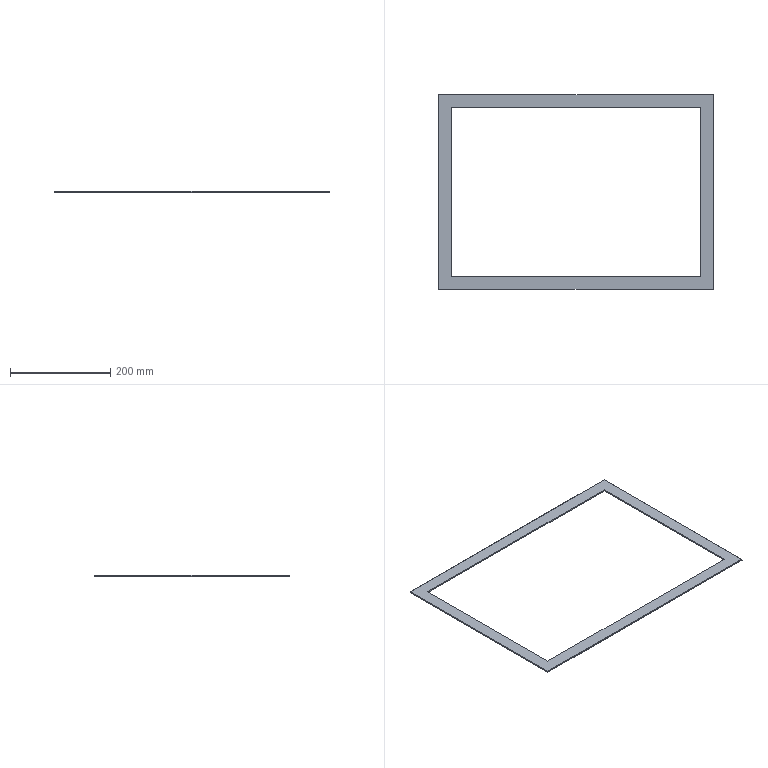Component | SolidWorks | LeftDoorPanelAssembly-1_WaterproofRubberStrip-1 | 1 solid | 18 faces | box 547.1 x 388.6 x 2.5 mm | volume 110544 mm3 | plane 18
build123d program:
from build123d import *

# Parameters (mm, degrees)
SKETCH1_W           = 547.1
SKETCH1_H           = 388.6
SKETCH1_W_2         = 497.1
SKETCH1_H_2         = 338.6
BOSS_EXTRUDE1_DEPTH = 2.5
CHAMFER1_SIZE       = 0.3


with BuildPart() as part:
    # Sketch1 → Boss-Extrude1 (new body)
    with BuildSketch(Plane.XY):
        Rectangle(SKETCH1_W, SKETCH1_H)
        Rectangle(SKETCH1_W_2, SKETCH1_H_2, mode=Mode.SUBTRACT)
    extrude(amount=BOSS_EXTRUDE1_DEPTH)

    # Chamfer1
    chamfer1_edges = [part.edges().sort_by_distance(p)[0] for p in [
        (273.55, 0, 2.5),
        (0, 194.3, 2.5),
        (-273.55, 0, 2.5),
        (0, 194.3, 0),
        (273.55, 0, 0),
        (0, -194.3, 0),
        (-273.55, 0, 0),
        (0, -194.3, 2.5),
    ]]
    chamfer(chamfer1_edges, length=CHAMFER1_SIZE)


solid = part.part

# Placed as in the assembly
solid = solid.moved(Location((235.358, 13.542, -71.9), (0, 0, 0)))
STEP:
#1=COLOUR_RGB('',0.7922,0.8196,0.9333);
#2=FILL_AREA_STYLE_COLOUR('',#1);
#3=FILL_AREA_STYLE('',(#2));
#4=SURFACE_STYLE_FILL_AREA(#3);
#5=SURFACE_SIDE_STYLE('',(#4));
#6=SURFACE_STYLE_USAGE(.BOTH.,#5);
#7=PRESENTATION_STYLE_ASSIGNMENT((#6));
#8=CARTESIAN_POINT('',(-1.492,8.171,-2.831));
#9=VERTEX_POINT('',#8);
#10=CARTESIAN_POINT('',(20.024,8.171,-2.831));
#11=VERTEX_POINT('',#10);
#12=CARTESIAN_POINT('',(20.036,8.171,-2.831));
#13=DIRECTION('',(1.,0.,0.));
#14=VECTOR('',#13,39.37);
#15=LINE('',#12,#14);
#16=EDGE_CURVE('',#9,#11,#15,.T.);
#17=ORIENTED_EDGE('',*,*,#16,.T.);
#18=CARTESIAN_POINT('',(20.024,-7.105,-2.831));
#19=VERTEX_POINT('',#18);
#20=CARTESIAN_POINT('',(20.024,-7.116,-2.831));
#21=DIRECTION('',(0.,-1.,0.));
#22=VECTOR('',#21,39.37);
#23=LINE('',#20,#22);
#24=EDGE_CURVE('',#11,#19,#23,.T.);
#25=ORIENTED_EDGE('',*,*,#24,.T.);
#26=CARTESIAN_POINT('',(-1.492,-7.105,-2.831));
#27=VERTEX_POINT('',#26);
#28=CARTESIAN_POINT('',(-1.504,-7.105,-2.831));
#29=DIRECTION('',(-1.,-0.,-0.));
#30=VECTOR('',#29,39.37);
#31=LINE('',#28,#30);
#32=EDGE_CURVE('',#19,#27,#31,.T.);
#33=ORIENTED_EDGE('',*,*,#32,.T.);
#34=CARTESIAN_POINT('',(-1.492,8.183,-2.831));
#35=DIRECTION('',(-0.,1.,-0.));
#36=VECTOR('',#35,39.37);
#37=LINE('',#34,#36);
#38=EDGE_CURVE('',#27,#9,#37,.T.);
#39=ORIENTED_EDGE('',*,*,#38,.T.);
#40=EDGE_LOOP('',(#17,#25,#33,#39));
#41=FACE_OUTER_BOUND('',#40,.T.);
#42=CARTESIAN_POINT('',(-0.5194,7.198,-2.831));
#43=VERTEX_POINT('',#42);
#44=CARTESIAN_POINT('',(19.052,7.198,-2.831));
#45=VERTEX_POINT('',#44);
#46=CARTESIAN_POINT('',(-0.5194,7.198,-2.831));
#47=DIRECTION('',(1.,0.,0.));
#48=VECTOR('',#47,39.37);
#49=LINE('',#46,#48);
#50=EDGE_CURVE('',#43,#45,#49,.T.);
#51=ORIENTED_EDGE('',*,*,#50,.F.);
#52=CARTESIAN_POINT('',(-0.5194,-6.132,-2.831));
#53=VERTEX_POINT('',#52);
#54=CARTESIAN_POINT('',(-0.5194,-6.132,-2.831));
#55=DIRECTION('',(-0.,1.,-0.));
#56=VECTOR('',#55,39.37);
#57=LINE('',#54,#56);
#58=EDGE_CURVE('',#53,#43,#57,.T.);
#59=ORIENTED_EDGE('',*,*,#58,.F.);
#60=CARTESIAN_POINT('',(19.052,-6.132,-2.831));
#61=VERTEX_POINT('',#60);
#62=CARTESIAN_POINT('',(-0.5194,-6.132,-2.831));
#63=DIRECTION('',(-1.,-0.,-0.));
#64=VECTOR('',#63,39.37);
#65=LINE('',#62,#64);
#66=EDGE_CURVE('',#61,#53,#65,.T.);
#67=ORIENTED_EDGE('',*,*,#66,.F.);
#68=CARTESIAN_POINT('',(19.052,-6.132,-2.831));
#69=DIRECTION('',(0.,-1.,0.));
#70=VECTOR('',#69,39.37);
#71=LINE('',#68,#70);
#72=EDGE_CURVE('',#45,#61,#71,.T.);
#73=ORIENTED_EDGE('',*,*,#72,.F.);
#74=EDGE_LOOP('',(#51,#59,#67,#73));
#75=FACE_BOUND('',#74,.T.);
#76=CARTESIAN_POINT('',(9.266,0.5331,-2.831));
#77=DIRECTION('',(0.,-0.,-1.));
#78=DIRECTION('',(-1.,-0.,-0.));
#79=AXIS2_PLACEMENT_3D('',#76,#77,#78);
#80=PLANE('',#79);
#81=ADVANCED_FACE('',(#41,#75),#80,.T.);
#82=CARTESIAN_POINT('',(-1.492,-7.105,-2.732));
#83=VERTEX_POINT('',#82);
#84=CARTESIAN_POINT('',(20.024,-7.105,-2.732));
#85=VERTEX_POINT('',#84);
#86=CARTESIAN_POINT('',(9.266,-7.105,-2.732));
#87=DIRECTION('',(1.,0.,0.));
#88=VECTOR('',#87,39.37);
#89=LINE('',#86,#88);
#90=EDGE_CURVE('',#83,#85,#89,.T.);
#91=ORIENTED_EDGE('',*,*,#90,.T.);
#92=CARTESIAN_POINT('',(20.024,8.171,-2.732));
#93=VERTEX_POINT('',#92);
#94=CARTESIAN_POINT('',(20.024,0.5331,-2.732));
#95=DIRECTION('',(-0.,1.,-0.));
#96=VECTOR('',#95,39.37);
#97=LINE('',#94,#96);
#98=EDGE_CURVE('',#85,#93,#97,.T.);
#99=ORIENTED_EDGE('',*,*,#98,.T.);
#100=CARTESIAN_POINT('',(-1.492,8.171,-2.732));
#101=VERTEX_POINT('',#100);
#102=CARTESIAN_POINT('',(9.266,8.171,-2.732));
#103=DIRECTION('',(-1.,-0.,-0.));
#104=VECTOR('',#103,39.37);
#105=LINE('',#102,#104);
#106=EDGE_CURVE('',#93,#101,#105,.T.);
#107=ORIENTED_EDGE('',*,*,#106,.T.);
#108=CARTESIAN_POINT('',(-1.492,0.5331,-2.732));
#109=DIRECTION('',(0.,-1.,0.));
#110=VECTOR('',#109,39.37);
#111=LINE('',#108,#110);
#112=EDGE_CURVE('',#101,#83,#111,.T.);
#113=ORIENTED_EDGE('',*,*,#112,.T.);
#114=EDGE_LOOP('',(#91,#99,#107,#113));
#115=FACE_OUTER_BOUND('',#114,.T.);
#116=CARTESIAN_POINT('',(-0.5194,-6.132,-2.732));
#117=VERTEX_POINT('',#116);
#118=CARTESIAN_POINT('',(-0.5194,7.198,-2.732));
#119=VERTEX_POINT('',#118);
#120=CARTESIAN_POINT('',(-0.5194,-6.132,-2.732));
#121=DIRECTION('',(-0.,1.,-0.));
#122=VECTOR('',#121,39.37);
#123=LINE('',#120,#122);
#124=EDGE_CURVE('',#117,#119,#123,.T.);
#125=ORIENTED_EDGE('',*,*,#124,.T.);
#126=CARTESIAN_POINT('',(19.052,7.198,-2.732));
#127=VERTEX_POINT('',#126);
#128=CARTESIAN_POINT('',(-0.5194,7.198,-2.732));
#129=DIRECTION('',(1.,0.,0.));
#130=VECTOR('',#129,39.37);
#131=LINE('',#128,#130);
#132=EDGE_CURVE('',#119,#127,#131,.T.);
#133=ORIENTED_EDGE('',*,*,#132,.T.);
#134=CARTESIAN_POINT('',(19.052,-6.132,-2.732));
#135=VERTEX_POINT('',#134);
#136=CARTESIAN_POINT('',(19.052,-6.132,-2.732));
#137=DIRECTION('',(0.,-1.,0.));
#138=VECTOR('',#137,39.37);
#139=LINE('',#136,#138);
#140=EDGE_CURVE('',#127,#135,#139,.T.);
#141=ORIENTED_EDGE('',*,*,#140,.T.);
#142=CARTESIAN_POINT('',(-0.5194,-6.132,-2.732));
#143=DIRECTION('',(-1.,-0.,-0.));
#144=VECTOR('',#143,39.37);
#145=LINE('',#142,#144);
#146=EDGE_CURVE('',#135,#117,#145,.T.);
#147=ORIENTED_EDGE('',*,*,#146,.T.);
#148=EDGE_LOOP('',(#125,#133,#141,#147));
#149=FACE_BOUND('',#148,.T.);
#150=CARTESIAN_POINT('',(9.266,0.5331,-2.732));
#151=DIRECTION('',(0.,-0.,-1.));
#152=DIRECTION('',(-1.,-0.,-0.));
#153=AXIS2_PLACEMENT_3D('',#150,#151,#152);
#154=PLANE('',#153);
#155=ADVANCED_FACE('',(#115,#149),#154,.F.);
#156=CARTESIAN_POINT('',(20.036,8.183,-2.819));
#157=VERTEX_POINT('',#156);
#158=CARTESIAN_POINT('',(20.036,8.183,-2.744));
#159=VERTEX_POINT('',#158);
#160=CARTESIAN_POINT('',(20.036,8.183,-2.831));
#161=DIRECTION('',(-0.,0.,1.));
#162=VECTOR('',#161,39.37);
#163=LINE('',#160,#162);
#164=EDGE_CURVE('',#157,#159,#163,.T.);
#165=ORIENTED_EDGE('',*,*,#164,.T.);
#166=CARTESIAN_POINT('',(20.036,-7.116,-2.744));
#167=VERTEX_POINT('',#166);
#168=CARTESIAN_POINT('',(20.036,-7.116,-2.744));
#169=DIRECTION('',(0.,-1.,0.));
#170=VECTOR('',#169,39.37);
#171=LINE('',#168,#170);
#172=EDGE_CURVE('',#159,#167,#171,.T.);
#173=ORIENTED_EDGE('',*,*,#172,.T.);
#174=CARTESIAN_POINT('',(20.036,-7.116,-2.819));
#175=VERTEX_POINT('',#174);
#176=CARTESIAN_POINT('',(20.036,-7.116,-2.831));
#177=DIRECTION('',(-0.,0.,1.));
#178=VECTOR('',#177,39.37);
#179=LINE('',#176,#178);
#180=EDGE_CURVE('',#175,#167,#179,.T.);
#181=ORIENTED_EDGE('',*,*,#180,.F.);
#182=CARTESIAN_POINT('',(20.036,8.183,-2.819));
#183=DIRECTION('',(-0.,1.,-0.));
#184=VECTOR('',#183,39.37);
#185=LINE('',#182,#184);
#186=EDGE_CURVE('',#175,#157,#185,.T.);
#187=ORIENTED_EDGE('',*,*,#186,.T.);
#188=EDGE_LOOP('',(#165,#173,#181,#187));
#189=FACE_OUTER_BOUND('',#188,.T.);
#190=CARTESIAN_POINT('',(20.036,-7.116,-2.831));
#191=DIRECTION('',(-1.,-0.,-0.));
#192=DIRECTION('',(-0.,0.,1.));
#193=AXIS2_PLACEMENT_3D('',#190,#191,#192);
#194=PLANE('',#193);
#195=ADVANCED_FACE('',(#189),#194,.F.);
#196=ORIENTED_EDGE('',*,*,#180,.T.);
#197=CARTESIAN_POINT('',(-1.504,-7.116,-2.744));
#198=VERTEX_POINT('',#197);
#199=CARTESIAN_POINT('',(-1.504,-7.116,-2.744));
#200=DIRECTION('',(-1.,-0.,-0.));
#201=VECTOR('',#200,39.37);
#202=LINE('',#199,#201);
#203=EDGE_CURVE('',#167,#198,#202,.T.);
#204=ORIENTED_EDGE('',*,*,#203,.T.);
#205=CARTESIAN_POINT('',(-1.504,-7.116,-2.819));
#206=VERTEX_POINT('',#205);
#207=CARTESIAN_POINT('',(-1.504,-7.116,-2.831));
#208=DIRECTION('',(-0.,0.,1.));
#209=VECTOR('',#208,39.37);
#210=LINE('',#207,#209);
#211=EDGE_CURVE('',#206,#198,#210,.T.);
#212=ORIENTED_EDGE('',*,*,#211,.F.);
#213=CARTESIAN_POINT('',(20.036,-7.116,-2.819));
#214=DIRECTION('',(1.,0.,0.));
#215=VECTOR('',#214,39.37);
#216=LINE('',#213,#215);
#217=EDGE_CURVE('',#206,#175,#216,.T.);
#218=ORIENTED_EDGE('',*,*,#217,.T.);
#219=EDGE_LOOP('',(#196,#204,#212,#218));
#220=FACE_OUTER_BOUND('',#219,.T.);
#221=CARTESIAN_POINT('',(-1.504,-7.116,-2.831));
#222=DIRECTION('',(-0.,1.,-0.));
#223=DIRECTION('',(1.,0.,0.));
#224=AXIS2_PLACEMENT_3D('',#221,#222,#223);
#225=PLANE('',#224);
#226=ADVANCED_FACE('',(#220),#225,.F.);
#227=ORIENTED_EDGE('',*,*,#211,.T.);
#228=CARTESIAN_POINT('',(-1.504,8.183,-2.744));
#229=VERTEX_POINT('',#228);
#230=CARTESIAN_POINT('',(-1.504,-7.116,-2.744));
#231=DIRECTION('',(-0.,1.,-0.));
#232=VECTOR('',#231,39.37);
#233=LINE('',#230,#232);
#234=EDGE_CURVE('',#198,#229,#233,.T.);
#235=ORIENTED_EDGE('',*,*,#234,.T.);
#236=CARTESIAN_POINT('',(-1.504,8.183,-2.819));
#237=VERTEX_POINT('',#236);
#238=CARTESIAN_POINT('',(-1.504,8.183,-2.831));
#239=DIRECTION('',(-0.,0.,1.));
#240=VECTOR('',#239,39.37);
#241=LINE('',#238,#240);
#242=EDGE_CURVE('',#237,#229,#241,.T.);
#243=ORIENTED_EDGE('',*,*,#242,.F.);
#244=CARTESIAN_POINT('',(-1.504,-7.116,-2.819));
#245=DIRECTION('',(0.,-1.,0.));
#246=VECTOR('',#245,39.37);
#247=LINE('',#244,#246);
#248=EDGE_CURVE('',#237,#206,#247,.T.);
#249=ORIENTED_EDGE('',*,*,#248,.T.);
#250=EDGE_LOOP('',(#227,#235,#243,#249));
#251=FACE_OUTER_BOUND('',#250,.T.);
#252=CARTESIAN_POINT('',(-1.504,-7.116,-2.831));
#253=DIRECTION('',(1.,0.,0.));
#254=DIRECTION('',(0.,-0.,-1.));
#255=AXIS2_PLACEMENT_3D('',#252,#253,#254);
#256=PLANE('',#255);
#257=ADVANCED_FACE('',(#251),#256,.F.);
#258=ORIENTED_EDGE('',*,*,#242,.T.);
#259=CARTESIAN_POINT('',(-1.504,8.183,-2.744));
#260=DIRECTION('',(1.,0.,0.));
#261=VECTOR('',#260,39.37);
#262=LINE('',#259,#261);
#263=EDGE_CURVE('',#229,#159,#262,.T.);
#264=ORIENTED_EDGE('',*,*,#263,.T.);
#265=ORIENTED_EDGE('',*,*,#164,.F.);
#266=CARTESIAN_POINT('',(-1.504,8.183,-2.819));
#267=DIRECTION('',(-1.,-0.,-0.));
#268=VECTOR('',#267,39.37);
#269=LINE('',#266,#268);
#270=EDGE_CURVE('',#157,#237,#269,.T.);
#271=ORIENTED_EDGE('',*,*,#270,.T.);
#272=EDGE_LOOP('',(#258,#264,#265,#271));
#273=FACE_OUTER_BOUND('',#272,.T.);
#274=CARTESIAN_POINT('',(-1.504,8.183,-2.831));
#275=DIRECTION('',(0.,-1.,0.));
#276=DIRECTION('',(-1.,-0.,-0.));
#277=AXIS2_PLACEMENT_3D('',#274,#275,#276);
#278=PLANE('',#277);
#279=ADVANCED_FACE('',(#273),#278,.F.);
#280=ORIENTED_EDGE('',*,*,#124,.F.);
#281=CARTESIAN_POINT('',(-0.5194,-6.132,-2.831));
#282=DIRECTION('',(-0.,0.,1.));
#283=VECTOR('',#282,39.37);
#284=LINE('',#281,#283);
#285=EDGE_CURVE('',#53,#117,#284,.T.);
#286=ORIENTED_EDGE('',*,*,#285,.F.);
#287=ORIENTED_EDGE('',*,*,#58,.T.);
#288=CARTESIAN_POINT('',(-0.5194,7.198,-2.831));
#289=DIRECTION('',(-0.,0.,1.));
#290=VECTOR('',#289,39.37);
#291=LINE('',#288,#290);
#292=EDGE_CURVE('',#43,#119,#291,.T.);
#293=ORIENTED_EDGE('',*,*,#292,.T.);
#294=EDGE_LOOP('',(#280,#286,#287,#293));
#295=FACE_OUTER_BOUND('',#294,.T.);
#296=CARTESIAN_POINT('',(-0.5194,-6.132,-2.831));
#297=DIRECTION('',(1.,0.,0.));
#298=DIRECTION('',(0.,-0.,-1.));
#299=AXIS2_PLACEMENT_3D('',#296,#297,#298);
#300=PLANE('',#299);
#301=ADVANCED_FACE('',(#295),#300,.T.);
#302=ORIENTED_EDGE('',*,*,#132,.F.);
#303=ORIENTED_EDGE('',*,*,#292,.F.);
#304=ORIENTED_EDGE('',*,*,#50,.T.);
#305=CARTESIAN_POINT('',(19.052,7.198,-2.831));
#306=DIRECTION('',(-0.,0.,1.));
#307=VECTOR('',#306,39.37);
#308=LINE('',#305,#307);
#309=EDGE_CURVE('',#45,#127,#308,.T.);
#310=ORIENTED_EDGE('',*,*,#309,.T.);
#311=EDGE_LOOP('',(#302,#303,#304,#310));
#312=FACE_OUTER_BOUND('',#311,.T.);
#313=CARTESIAN_POINT('',(-0.5194,7.198,-2.831));
#314=DIRECTION('',(0.,-1.,0.));
#315=DIRECTION('',(-1.,-0.,-0.));
#316=AXIS2_PLACEMENT_3D('',#313,#314,#315);
#317=PLANE('',#316);
#318=ADVANCED_FACE('',(#312),#317,.T.);
#319=ORIENTED_EDGE('',*,*,#140,.F.);
#320=ORIENTED_EDGE('',*,*,#309,.F.);
#321=ORIENTED_EDGE('',*,*,#72,.T.);
#322=CARTESIAN_POINT('',(19.052,-6.132,-2.831));
#323=DIRECTION('',(-0.,0.,1.));
#324=VECTOR('',#323,39.37);
#325=LINE('',#322,#324);
#326=EDGE_CURVE('',#61,#135,#325,.T.);
#327=ORIENTED_EDGE('',*,*,#326,.T.);
#328=EDGE_LOOP('',(#319,#320,#321,#327));
#329=FACE_OUTER_BOUND('',#328,.T.);
#330=CARTESIAN_POINT('',(19.052,-6.132,-2.831));
#331=DIRECTION('',(-1.,-0.,-0.));
#332=DIRECTION('',(-0.,1.,-0.));
#333=AXIS2_PLACEMENT_3D('',#330,#331,#332);
#334=PLANE('',#333);
#335=ADVANCED_FACE('',(#329),#334,.T.);
#336=ORIENTED_EDGE('',*,*,#146,.F.);
#337=ORIENTED_EDGE('',*,*,#326,.F.);
#338=ORIENTED_EDGE('',*,*,#66,.T.);
#339=ORIENTED_EDGE('',*,*,#285,.T.);
#340=EDGE_LOOP('',(#336,#337,#338,#339));
#341=FACE_OUTER_BOUND('',#340,.T.);
#342=CARTESIAN_POINT('',(-0.5194,-6.132,-2.831));
#343=DIRECTION('',(-0.,1.,-0.));
#344=DIRECTION('',(1.,0.,0.));
#345=AXIS2_PLACEMENT_3D('',#342,#343,#344);
#346=PLANE('',#345);
#347=ADVANCED_FACE('',(#341),#346,.T.);
#348=CARTESIAN_POINT('',(-1.504,-7.116,-2.744));
#349=DIRECTION('',(-0.5774,-0.5774,-0.5774));
#350=VECTOR('',#349,39.37);
#351=LINE('',#348,#350);
#352=EDGE_CURVE('',#83,#198,#351,.T.);
#353=ORIENTED_EDGE('',*,*,#352,.F.);
#354=ORIENTED_EDGE('',*,*,#112,.F.);
#355=CARTESIAN_POINT('',(-1.504,8.183,-2.744));
#356=DIRECTION('',(0.5774,-0.5774,0.5774));
#357=VECTOR('',#356,39.37);
#358=LINE('',#355,#357);
#359=EDGE_CURVE('',#229,#101,#358,.T.);
#360=ORIENTED_EDGE('',*,*,#359,.F.);
#361=ORIENTED_EDGE('',*,*,#234,.F.);
#362=EDGE_LOOP('',(#353,#354,#360,#361));
#363=FACE_OUTER_BOUND('',#362,.T.);
#364=CARTESIAN_POINT('',(-1.504,-7.116,-2.744));
#365=DIRECTION('',(0.7071,-0.,-0.7071));
#366=DIRECTION('',(-0.,1.,-0.));
#367=AXIS2_PLACEMENT_3D('',#364,#365,#366);
#368=PLANE('',#367);
#369=ADVANCED_FACE('',(#363),#368,.F.);
#370=ORIENTED_EDGE('',*,*,#359,.T.);
#371=ORIENTED_EDGE('',*,*,#106,.F.);
#372=CARTESIAN_POINT('',(12.856,1.003,4.436));
#373=DIRECTION('',(-0.5774,-0.5774,0.5774));
#374=VECTOR('',#373,39.37);
#375=LINE('',#372,#374);
#376=EDGE_CURVE('',#159,#93,#375,.T.);
#377=ORIENTED_EDGE('',*,*,#376,.F.);
#378=ORIENTED_EDGE('',*,*,#263,.F.);
#379=EDGE_LOOP('',(#370,#371,#377,#378));
#380=FACE_OUTER_BOUND('',#379,.T.);
#381=CARTESIAN_POINT('',(-1.504,8.183,-2.744));
#382=DIRECTION('',(0.,-0.7071,-0.7071));
#383=DIRECTION('',(1.,0.,0.));
#384=AXIS2_PLACEMENT_3D('',#381,#382,#383);
#385=PLANE('',#384);
#386=ADVANCED_FACE('',(#380),#385,.F.);
#387=ORIENTED_EDGE('',*,*,#352,.T.);
#388=ORIENTED_EDGE('',*,*,#203,.F.);
#389=CARTESIAN_POINT('',(12.856,0.06332,4.436));
#390=DIRECTION('',(0.5774,-0.5774,-0.5774));
#391=VECTOR('',#390,39.37);
#392=LINE('',#389,#391);
#393=EDGE_CURVE('',#85,#167,#392,.T.);
#394=ORIENTED_EDGE('',*,*,#393,.F.);
#395=ORIENTED_EDGE('',*,*,#90,.F.);
#396=EDGE_LOOP('',(#387,#388,#394,#395));
#397=FACE_OUTER_BOUND('',#396,.T.);
#398=CARTESIAN_POINT('',(-1.504,-7.116,-2.744));
#399=DIRECTION('',(0.,0.7071,-0.7071));
#400=DIRECTION('',(-1.,-0.,-0.));
#401=AXIS2_PLACEMENT_3D('',#398,#399,#400);
#402=PLANE('',#401);
#403=ADVANCED_FACE('',(#397),#402,.F.);
#404=ORIENTED_EDGE('',*,*,#376,.T.);
#405=ORIENTED_EDGE('',*,*,#98,.F.);
#406=ORIENTED_EDGE('',*,*,#393,.T.);
#407=ORIENTED_EDGE('',*,*,#172,.F.);
#408=EDGE_LOOP('',(#404,#405,#406,#407));
#409=FACE_OUTER_BOUND('',#408,.T.);
#410=CARTESIAN_POINT('',(20.036,-7.116,-2.744));
#411=DIRECTION('',(-0.7071,-0.,-0.7071));
#412=DIRECTION('',(0.,-1.,0.));
#413=AXIS2_PLACEMENT_3D('',#410,#411,#412);
#414=PLANE('',#413);
#415=ADVANCED_FACE('',(#409),#414,.F.);
#416=CARTESIAN_POINT('',(1.054,-4.559,-5.377));
#417=DIRECTION('',(0.5774,0.5774,-0.5774));
#418=VECTOR('',#417,39.37);
#419=LINE('',#416,#418);
#420=EDGE_CURVE('',#206,#27,#419,.T.);
#421=ORIENTED_EDGE('',*,*,#420,.F.);
#422=ORIENTED_EDGE('',*,*,#248,.F.);
#423=CARTESIAN_POINT('',(2.094,4.585,-6.417));
#424=DIRECTION('',(-0.5774,0.5774,0.5774));
#425=VECTOR('',#424,39.37);
#426=LINE('',#423,#425);
#427=EDGE_CURVE('',#9,#237,#426,.T.);
#428=ORIENTED_EDGE('',*,*,#427,.F.);
#429=ORIENTED_EDGE('',*,*,#38,.F.);
#430=EDGE_LOOP('',(#421,#422,#428,#429));
#431=FACE_OUTER_BOUND('',#430,.T.);
#432=CARTESIAN_POINT('',(-1.492,0.5331,-2.831));
#433=DIRECTION('',(-0.7071,-0.,-0.7071));
#434=DIRECTION('',(0.,-1.,0.));
#435=AXIS2_PLACEMENT_3D('',#432,#433,#434);
#436=PLANE('',#435);
#437=ADVANCED_FACE('',(#431),#436,.T.);
#438=ORIENTED_EDGE('',*,*,#427,.T.);
#439=ORIENTED_EDGE('',*,*,#270,.F.);
#440=CARTESIAN_POINT('',(16.438,4.585,-6.417));
#441=DIRECTION('',(0.5774,0.5774,0.5774));
#442=VECTOR('',#441,39.37);
#443=LINE('',#440,#442);
#444=EDGE_CURVE('',#11,#157,#443,.T.);
#445=ORIENTED_EDGE('',*,*,#444,.F.);
#446=ORIENTED_EDGE('',*,*,#16,.F.);
#447=EDGE_LOOP('',(#438,#439,#445,#446));
#448=FACE_OUTER_BOUND('',#447,.T.);
#449=CARTESIAN_POINT('',(9.266,8.171,-2.831));
#450=DIRECTION('',(0.,0.7071,-0.7071));
#451=DIRECTION('',(-1.,-0.,-0.));
#452=AXIS2_PLACEMENT_3D('',#449,#450,#451);
#453=PLANE('',#452);
#454=ADVANCED_FACE('',(#448),#453,.T.);
#455=ORIENTED_EDGE('',*,*,#420,.T.);
#456=ORIENTED_EDGE('',*,*,#32,.F.);
#457=CARTESIAN_POINT('',(16.438,-3.519,-6.417));
#458=DIRECTION('',(-0.5774,0.5774,-0.5774));
#459=VECTOR('',#458,39.37);
#460=LINE('',#457,#459);
#461=EDGE_CURVE('',#175,#19,#460,.T.);
#462=ORIENTED_EDGE('',*,*,#461,.F.);
#463=ORIENTED_EDGE('',*,*,#217,.F.);
#464=EDGE_LOOP('',(#455,#456,#462,#463));
#465=FACE_OUTER_BOUND('',#464,.T.);
#466=CARTESIAN_POINT('',(9.266,-7.105,-2.831));
#467=DIRECTION('',(0.,-0.7071,-0.7071));
#468=DIRECTION('',(1.,0.,0.));
#469=AXIS2_PLACEMENT_3D('',#466,#467,#468);
#470=PLANE('',#469);
#471=ADVANCED_FACE('',(#465),#470,.T.);
#472=ORIENTED_EDGE('',*,*,#444,.T.);
#473=ORIENTED_EDGE('',*,*,#186,.F.);
#474=ORIENTED_EDGE('',*,*,#461,.T.);
#475=ORIENTED_EDGE('',*,*,#24,.F.);
#476=EDGE_LOOP('',(#472,#473,#474,#475));
#477=FACE_OUTER_BOUND('',#476,.T.);
#478=CARTESIAN_POINT('',(20.024,0.5331,-2.831));
#479=DIRECTION('',(0.7071,-0.,-0.7071));
#480=DIRECTION('',(-0.,1.,-0.));
#481=AXIS2_PLACEMENT_3D('',#478,#479,#480);
#482=PLANE('',#481);
#483=ADVANCED_FACE('',(#477),#482,.T.);
#484=CLOSED_SHELL('',(#81,#155,#195,#226,#257,#279,#301,#318,#335,#347,#369,#386,#403,#415,#437,#454,#471,#483));
#485=MANIFOLD_SOLID_BREP('',#484);
#486=STYLED_ITEM('',(#7),#485);
#487=PRESENTATION_LAYER_ASSIGNMENT('','',(#486));
#488=(LENGTH_UNIT()NAMED_UNIT(*)SI_UNIT($,.METRE.));
#489=LENGTH_MEASURE_WITH_UNIT(LENGTH_MEASURE(0.0254),#488);
#490=DIMENSIONAL_EXPONENTS(1.,0.,0.,0.,0.,0.,0.);
#491=(CONVERSION_BASED_UNIT('',#489)LENGTH_UNIT()NAMED_UNIT(#490));
#492=UNCERTAINTY_MEASURE_WITH_UNIT(LENGTH_MEASURE(0.00001),#491,'','');
#493=(NAMED_UNIT(*)PLANE_ANGLE_UNIT()SI_UNIT($,.RADIAN.));
#494=(NAMED_UNIT(*)SI_UNIT($,.STERADIAN.)SOLID_ANGLE_UNIT());
#495=(GEOMETRIC_REPRESENTATION_CONTEXT(3)GLOBAL_UNCERTAINTY_ASSIGNED_CONTEXT((#492))GLOBAL_UNIT_ASSIGNED_CONTEXT((#491,#493,#494))REPRESENTATION_CONTEXT('',''));
#496=MECHANICAL_DESIGN_GEOMETRIC_PRESENTATION_REPRESENTATION('',(#486),#495);
#497=CARTESIAN_POINT('',(0.,0.,0.));
#498=DIRECTION('',(0.,0.,1.));
#499=DIRECTION('',(1.,0.,0.));
#500=AXIS2_PLACEMENT_3D('',#497,#498,#499);
#501=(LENGTH_UNIT()NAMED_UNIT(*)SI_UNIT($,.METRE.));
#502=LENGTH_MEASURE_WITH_UNIT(LENGTH_MEASURE(0.0254),#501);
#503=DIMENSIONAL_EXPONENTS(1.,0.,0.,0.,0.,0.,0.);
#504=(CONVERSION_BASED_UNIT('',#502)LENGTH_UNIT()NAMED_UNIT(#503));
#505=UNCERTAINTY_MEASURE_WITH_UNIT(LENGTH_MEASURE(0.00001),#504,'','');
#506=(NAMED_UNIT(*)PLANE_ANGLE_UNIT()SI_UNIT($,.RADIAN.));
#507=(NAMED_UNIT(*)SI_UNIT($,.STERADIAN.)SOLID_ANGLE_UNIT());
#508=(GEOMETRIC_REPRESENTATION_CONTEXT(3)GLOBAL_UNCERTAINTY_ASSIGNED_CONTEXT((#505))GLOBAL_UNIT_ASSIGNED_CONTEXT((#504,#506,#507))REPRESENTATION_CONTEXT('',''));
#509=ADVANCED_BREP_SHAPE_REPRESENTATION('',(#485,#500),#508);